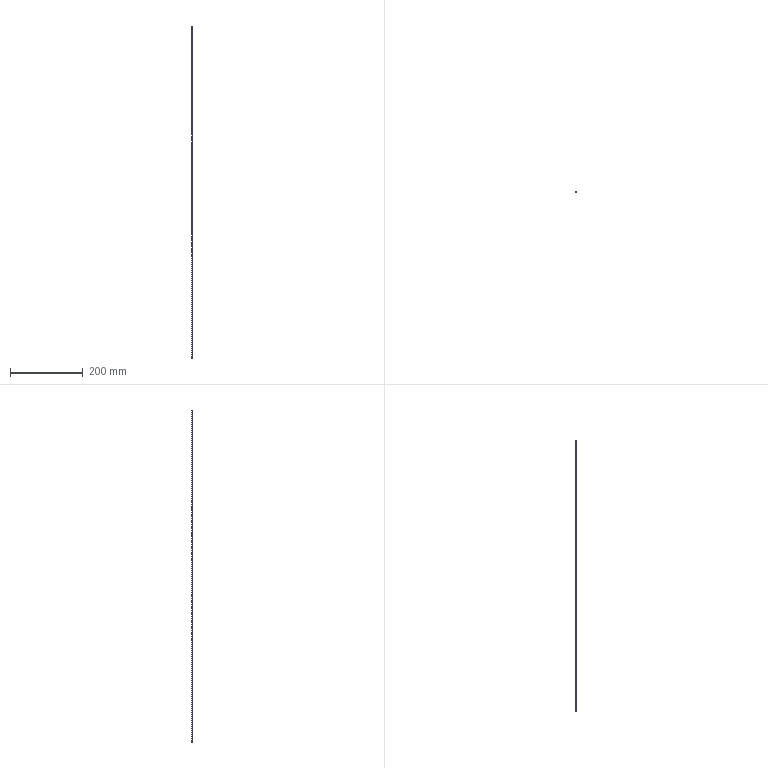Component | NX | CABLE | 1 solid | 3 faces | box 2 x 2 x 910 mm | volume 2859 mm3 | plane 2 | cylinder 1 | commonest cylinder face diameters 2 x1
STEP:
#1=CARTESIAN_POINT('',(0.,0.,0.));
#2=DIRECTION('',(0.,0.,1.));
#3=DIRECTION('',(1.,0.,0.));
#4=AXIS2_PLACEMENT_3D('',#1,#2,#3);
#5=CARTESIAN_POINT('',(35.,384.,339.346));
#6=VERTEX_POINT('',#5);
#7=CARTESIAN_POINT('',(34.,384.,339.346));
#8=DIRECTION('',(0.,-0.,1.));
#9=DIRECTION('',(1.,0.,-0.));
#10=AXIS2_PLACEMENT_3D('',#7,#8,#9);
#11=CIRCLE('',#10,1.);
#12=CARTESIAN_POINT('',(34.,384.,339.346));
#13=DIRECTION('',(-0.,0.,1.));
#14=DIRECTION('',(0.,1.,0.));
#15=AXIS2_PLACEMENT_3D('',#12,#13,#14);
#16=PLANE('',#15);
#17=CARTESIAN_POINT('',(0.,-0.));
#18=DIRECTION('',(0.,-1.));
#19=AXIS2_PLACEMENT_2D('',#17,#18);
#20=CIRCLE('',#19,1.);
#21=(GEOMETRIC_REPRESENTATION_CONTEXT(2)PARAMETRIC_REPRESENTATION_CONTEXT()REPRESENTATION_CONTEXT('',''));
#22=DEFINITIONAL_REPRESENTATION('',(#20),#21);
#23=PCURVE('',#16,#22);
#24=CARTESIAN_POINT('',(34.,384.,-570.654));
#25=DIRECTION('',(0.,0.,1.));
#26=DIRECTION('',(1.,0.,-0.));
#27=AXIS2_PLACEMENT_3D('',#24,#25,#26);
#28=CYLINDRICAL_SURFACE('',#27,1.);
#29=CARTESIAN_POINT('',(0.,910.));
#30=DIRECTION('',(1.,0.));
#31=VECTOR('',#30,1.);
#32=LINE('',#29,#31);
#33=(GEOMETRIC_REPRESENTATION_CONTEXT(2)PARAMETRIC_REPRESENTATION_CONTEXT()REPRESENTATION_CONTEXT('',''));
#34=DEFINITIONAL_REPRESENTATION('',(#32),#33);
#35=PCURVE('',#28,#34);
#36=SURFACE_CURVE('',#11,(#23,#35),.PCURVE_S1.);
#37=EDGE_CURVE('',#6,#6,#36,.T.);
#38=ORIENTED_EDGE('',*,*,#37,.T.);
#39=EDGE_LOOP('',(#38));
#40=FACE_BOUND('',#39,.T.);
#41=ADVANCED_FACE('',(#40),#16,.T.);
#42=CARTESIAN_POINT('',(35.,384.,-570.654));
#43=VERTEX_POINT('',#42);
#44=CARTESIAN_POINT('',(34.,384.,-570.654));
#45=DIRECTION('',(0.,-0.,-1.));
#46=DIRECTION('',(1.,-0.,0.));
#47=AXIS2_PLACEMENT_3D('',#44,#45,#46);
#48=CIRCLE('',#47,1.);
#49=CARTESIAN_POINT('',(34.,384.,-570.654));
#50=DIRECTION('',(0.,0.,1.));
#51=DIRECTION('',(0.,1.,-0.));
#52=AXIS2_PLACEMENT_3D('',#49,#50,#51);
#53=PLANE('',#52);
#54=CARTESIAN_POINT('',(0.,-1.));
#55=CARTESIAN_POINT('',(-1.732,-1.));
#56=CARTESIAN_POINT('',(-0.866,0.5));
#57=CARTESIAN_POINT('',(-0.,2.));
#58=CARTESIAN_POINT('',(0.866,0.5));
#59=CARTESIAN_POINT('',(1.732,-1.));
#60=CARTESIAN_POINT('',(0.,-1.));
#61=(BOUNDED_CURVE()B_SPLINE_CURVE(2,(#54,#55,#56,#57,#58,#59,#60),.UNSPECIFIED.,.T.,.F.)B_SPLINE_CURVE_WITH_KNOTS((1,2,2,2,2,1),(-2.094,0.,2.094,4.189,6.283,8.378),.UNSPECIFIED.)CURVE()GEOMETRIC_REPRESENTATION_ITEM()RATIONAL_B_SPLINE_CURVE((1.,0.5,1.,0.5,1.,0.5,1.))REPRESENTATION_ITEM(''));
#62=(GEOMETRIC_REPRESENTATION_CONTEXT(2)PARAMETRIC_REPRESENTATION_CONTEXT()REPRESENTATION_CONTEXT('',''));
#63=DEFINITIONAL_REPRESENTATION('',(#61),#62);
#64=PCURVE('',#53,#63);
#65=CARTESIAN_POINT('',(6.283,0.));
#66=DIRECTION('',(-1.,0.));
#67=VECTOR('',#66,1.);
#68=LINE('',#65,#67);
#69=(GEOMETRIC_REPRESENTATION_CONTEXT(2)PARAMETRIC_REPRESENTATION_CONTEXT()REPRESENTATION_CONTEXT('',''));
#70=DEFINITIONAL_REPRESENTATION('',(#68),#69);
#71=PCURVE('',#28,#70);
#72=SURFACE_CURVE('',#48,(#64,#71),.PCURVE_S1.);
#73=EDGE_CURVE('',#43,#43,#72,.T.);
#74=ORIENTED_EDGE('',*,*,#73,.T.);
#75=EDGE_LOOP('',(#74));
#76=FACE_BOUND('',#75,.T.);
#77=ADVANCED_FACE('',(#76),#53,.F.);
#78=ORIENTED_EDGE('',*,*,#73,.F.);
#79=CARTESIAN_POINT('',(35.,384.,-570.654));
#80=CARTESIAN_POINT('',(35.,384.,339.346));
#81=B_SPLINE_CURVE_WITH_KNOTS('',1,(#79,#80),.UNSPECIFIED.,.F.,.F.,(2,2),(0.,910.),.PIECEWISE_BEZIER_KNOTS.);
#82=CARTESIAN_POINT('',(6.283,0.));
#83=DIRECTION('',(0.,1.));
#84=VECTOR('',#83,1.);
#85=LINE('',#82,#84);
#86=(GEOMETRIC_REPRESENTATION_CONTEXT(2)PARAMETRIC_REPRESENTATION_CONTEXT()REPRESENTATION_CONTEXT('',''));
#87=DEFINITIONAL_REPRESENTATION('',(#85),#86);
#88=PCURVE('',#28,#87);
#89=CARTESIAN_POINT('',(0.,0.));
#90=DIRECTION('',(0.,1.));
#91=VECTOR('',#90,1.);
#92=LINE('',#89,#91);
#93=(GEOMETRIC_REPRESENTATION_CONTEXT(2)PARAMETRIC_REPRESENTATION_CONTEXT()REPRESENTATION_CONTEXT('',''));
#94=DEFINITIONAL_REPRESENTATION('',(#92),#93);
#95=PCURVE('',#28,#94);
#96=SEAM_CURVE('',#81,(#88,#95),.PCURVE_S1.);
#97=EDGE_CURVE('',#43,#6,#96,.T.);
#98=ORIENTED_EDGE('',*,*,#97,.T.);
#99=ORIENTED_EDGE('',*,*,#37,.F.);
#100=ORIENTED_EDGE('',*,*,#97,.F.);
#101=EDGE_LOOP('',(#78,#98,#99,#100));
#102=FACE_BOUND('',#101,.T.);
#103=ADVANCED_FACE('',(#102),#28,.T.);
#104=CLOSED_SHELL('',(#41,#77,#103));
#105=MANIFOLD_SOLID_BREP('',#104);
#106=(LENGTH_UNIT()NAMED_UNIT(*)SI_UNIT(.MILLI.,.METRE.));
#107=UNCERTAINTY_MEASURE_WITH_UNIT(LENGTH_MEASURE(0.00001),#106,'','');
#108=(NAMED_UNIT(*)PLANE_ANGLE_UNIT()SI_UNIT($,.RADIAN.));
#109=(NAMED_UNIT(*)SI_UNIT($,.STERADIAN.)SOLID_ANGLE_UNIT());
#110=(GEOMETRIC_REPRESENTATION_CONTEXT(3)GLOBAL_UNCERTAINTY_ASSIGNED_CONTEXT((#107))GLOBAL_UNIT_ASSIGNED_CONTEXT((#106,#108,#109))REPRESENTATION_CONTEXT('',''));
#111=ADVANCED_BREP_SHAPE_REPRESENTATION('',(#4,#105),#110);